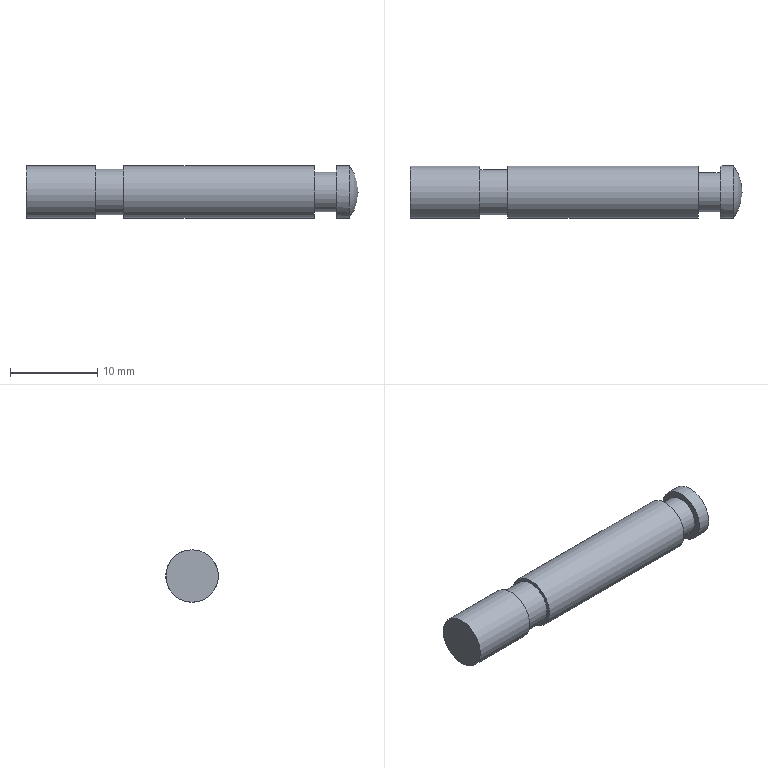Component | NX | SUPPORT_STUD | 1 solid | 11 faces | box 38 x 6 x 6 mm | volume 1007 mm3 | cylinder 5 | plane 5 | sphere 1 | commonest cylinder face diameters 6 x3 4.5 x1 5.188 x1
STEP:
#1=CARTESIAN_POINT('',(0.,0.,0.));
#2=DIRECTION('',(0.,0.,1.));
#3=DIRECTION('',(1.,0.,0.));
#4=AXIS2_PLACEMENT_3D('',#1,#2,#3);
#5=CARTESIAN_POINT('',(-18.8,-52.,-54.));
#6=VERTEX_POINT('',#5);
#7=CARTESIAN_POINT('',(-18.8,-52.,-57.));
#8=DIRECTION('',(1.,0.,-0.));
#9=DIRECTION('',(0.,0.,1.));
#10=AXIS2_PLACEMENT_3D('',#7,#8,#9);
#11=CIRCLE('',#10,3.);
#12=CARTESIAN_POINT('',(-30.,-52.,-57.));
#13=DIRECTION('',(1.,0.,0.));
#14=DIRECTION('',(0.,0.,1.));
#15=AXIS2_PLACEMENT_3D('',#12,#13,#14);
#16=CYLINDRICAL_SURFACE('',#15,3.);
#17=CARTESIAN_POINT('',(0.,11.2));
#18=DIRECTION('',(1.,0.));
#19=VECTOR('',#18,1.);
#20=LINE('',#17,#19);
#21=(GEOMETRIC_REPRESENTATION_CONTEXT(2)PARAMETRIC_REPRESENTATION_CONTEXT()REPRESENTATION_CONTEXT('',''));
#22=DEFINITIONAL_REPRESENTATION('',(#20),#21);
#23=PCURVE('',#16,#22);
#24=CARTESIAN_POINT('',(-18.8,-52.,-57.));
#25=DIRECTION('',(1.,0.,-0.));
#26=DIRECTION('',(0.,-1.,0.));
#27=AXIS2_PLACEMENT_3D('',#24,#25,#26);
#28=PLANE('',#27);
#29=CARTESIAN_POINT('',(0.,0.));
#30=DIRECTION('',(0.,-1.));
#31=AXIS2_PLACEMENT_2D('',#29,#30);
#32=CIRCLE('',#31,3.);
#33=(GEOMETRIC_REPRESENTATION_CONTEXT(2)PARAMETRIC_REPRESENTATION_CONTEXT()REPRESENTATION_CONTEXT('',''));
#34=DEFINITIONAL_REPRESENTATION('',(#32),#33);
#35=PCURVE('',#28,#34);
#36=SURFACE_CURVE('',#11,(#23,#35),.PCURVE_S1.);
#37=EDGE_CURVE('',#6,#6,#36,.T.);
#38=ORIENTED_EDGE('',*,*,#37,.T.);
#39=CARTESIAN_POINT('',(3.,-52.,-54.));
#40=VERTEX_POINT('',#39);
#41=CARTESIAN_POINT('',(-18.8,-52.,-54.));
#42=CARTESIAN_POINT('',(3.,-52.,-54.));
#43=B_SPLINE_CURVE_WITH_KNOTS('',1,(#41,#42),.UNSPECIFIED.,.F.,.F.,(2,2),(11.2,33.),.PIECEWISE_BEZIER_KNOTS.);
#44=CARTESIAN_POINT('',(6.283,0.));
#45=DIRECTION('',(0.,1.));
#46=VECTOR('',#45,1.);
#47=LINE('',#44,#46);
#48=(GEOMETRIC_REPRESENTATION_CONTEXT(2)PARAMETRIC_REPRESENTATION_CONTEXT()REPRESENTATION_CONTEXT('',''));
#49=DEFINITIONAL_REPRESENTATION('',(#47),#48);
#50=PCURVE('',#16,#49);
#51=CARTESIAN_POINT('',(0.,0.));
#52=DIRECTION('',(0.,1.));
#53=VECTOR('',#52,1.);
#54=LINE('',#51,#53);
#55=(GEOMETRIC_REPRESENTATION_CONTEXT(2)PARAMETRIC_REPRESENTATION_CONTEXT()REPRESENTATION_CONTEXT('',''));
#56=DEFINITIONAL_REPRESENTATION('',(#54),#55);
#57=PCURVE('',#16,#56);
#58=SEAM_CURVE('',#43,(#50,#57),.PCURVE_S1.);
#59=EDGE_CURVE('',#6,#40,#58,.T.);
#60=ORIENTED_EDGE('',*,*,#59,.T.);
#61=CARTESIAN_POINT('',(3.,-52.,-57.));
#62=DIRECTION('',(1.,0.,0.));
#63=DIRECTION('',(0.,0.,1.));
#64=AXIS2_PLACEMENT_3D('',#61,#62,#63);
#65=CIRCLE('',#64,3.);
#66=CARTESIAN_POINT('',(0.,33.));
#67=DIRECTION('',(1.,0.));
#68=VECTOR('',#67,1.);
#69=LINE('',#66,#68);
#70=(GEOMETRIC_REPRESENTATION_CONTEXT(2)PARAMETRIC_REPRESENTATION_CONTEXT()REPRESENTATION_CONTEXT('',''));
#71=DEFINITIONAL_REPRESENTATION('',(#69),#70);
#72=PCURVE('',#16,#71);
#73=CARTESIAN_POINT('',(3.,-52.,-57.));
#74=DIRECTION('',(1.,0.,0.));
#75=DIRECTION('',(0.,0.,1.));
#76=AXIS2_PLACEMENT_3D('',#73,#74,#75);
#77=PLANE('',#76);
#78=CARTESIAN_POINT('',(0.,0.));
#79=DIRECTION('',(1.,0.));
#80=AXIS2_PLACEMENT_2D('',#78,#79);
#81=CIRCLE('',#80,3.);
#82=(GEOMETRIC_REPRESENTATION_CONTEXT(2)PARAMETRIC_REPRESENTATION_CONTEXT()REPRESENTATION_CONTEXT('',''));
#83=DEFINITIONAL_REPRESENTATION('',(#81),#82);
#84=PCURVE('',#77,#83);
#85=SURFACE_CURVE('',#65,(#72,#84),.PCURVE_S1.);
#86=EDGE_CURVE('',#40,#40,#85,.T.);
#87=ORIENTED_EDGE('',*,*,#86,.F.);
#88=ORIENTED_EDGE('',*,*,#59,.F.);
#89=EDGE_LOOP('',(#38,#60,#87,#88));
#90=FACE_BOUND('',#89,.T.);
#91=ADVANCED_FACE('',(#90),#16,.T.);
#92=CARTESIAN_POINT('',(3.,-52.,-54.75));
#93=VERTEX_POINT('',#92);
#94=CARTESIAN_POINT('',(3.,-52.,-57.));
#95=DIRECTION('',(-1.,0.,0.));
#96=DIRECTION('',(0.,0.,1.));
#97=AXIS2_PLACEMENT_3D('',#94,#95,#96);
#98=CIRCLE('',#97,2.25);
#99=CARTESIAN_POINT('',(2.25,0.));
#100=CARTESIAN_POINT('',(2.25,-3.897));
#101=CARTESIAN_POINT('',(-1.125,-1.949));
#102=CARTESIAN_POINT('',(-4.5,-0.));
#103=CARTESIAN_POINT('',(-1.125,1.949));
#104=CARTESIAN_POINT('',(2.25,3.897));
#105=CARTESIAN_POINT('',(2.25,0.));
#106=(BOUNDED_CURVE()B_SPLINE_CURVE(2,(#99,#100,#101,#102,#103,#104,#105),.UNSPECIFIED.,.T.,.F.)B_SPLINE_CURVE_WITH_KNOTS((1,2,2,2,2,1),(-2.094,0.,2.094,4.189,6.283,8.378),.UNSPECIFIED.)CURVE()GEOMETRIC_REPRESENTATION_ITEM()RATIONAL_B_SPLINE_CURVE((1.,0.5,1.,0.5,1.,0.5,1.))REPRESENTATION_ITEM(''));
#107=(GEOMETRIC_REPRESENTATION_CONTEXT(2)PARAMETRIC_REPRESENTATION_CONTEXT()REPRESENTATION_CONTEXT('',''));
#108=DEFINITIONAL_REPRESENTATION('',(#106),#107);
#109=PCURVE('',#77,#108);
#110=CARTESIAN_POINT('',(-3.75,-52.,-57.));
#111=DIRECTION('',(1.,0.,0.));
#112=DIRECTION('',(0.,0.,1.));
#113=AXIS2_PLACEMENT_3D('',#110,#111,#112);
#114=CYLINDRICAL_SURFACE('',#113,2.25);
#115=CARTESIAN_POINT('',(6.283,6.75));
#116=DIRECTION('',(-1.,0.));
#117=VECTOR('',#116,1.);
#118=LINE('',#115,#117);
#119=(GEOMETRIC_REPRESENTATION_CONTEXT(2)PARAMETRIC_REPRESENTATION_CONTEXT()REPRESENTATION_CONTEXT('',''));
#120=DEFINITIONAL_REPRESENTATION('',(#118),#119);
#121=PCURVE('',#114,#120);
#122=SURFACE_CURVE('',#98,(#109,#121),.PCURVE_S1.);
#123=EDGE_CURVE('',#93,#93,#122,.T.);
#124=ORIENTED_EDGE('',*,*,#123,.T.);
#125=EDGE_LOOP('',(#124));
#126=FACE_BOUND('',#125,.T.);
#127=ORIENTED_EDGE('',*,*,#86,.T.);
#128=EDGE_LOOP('',(#127));
#129=FACE_BOUND('',#128,.T.);
#130=ADVANCED_FACE('',(#126,#129),#77,.T.);
#131=CARTESIAN_POINT('',(5.5,-52.,-54.75));
#132=VERTEX_POINT('',#131);
#133=CARTESIAN_POINT('',(5.5,-52.,-57.));
#134=DIRECTION('',(-1.,0.,0.));
#135=DIRECTION('',(0.,0.,1.));
#136=AXIS2_PLACEMENT_3D('',#133,#134,#135);
#137=CIRCLE('',#136,2.25);
#138=CARTESIAN_POINT('',(5.5,-52.,-57.));
#139=DIRECTION('',(1.,0.,0.));
#140=DIRECTION('',(0.,0.,1.));
#141=AXIS2_PLACEMENT_3D('',#138,#139,#140);
#142=PLANE('',#141);
#143=CARTESIAN_POINT('',(2.25,0.));
#144=CARTESIAN_POINT('',(2.25,-3.897));
#145=CARTESIAN_POINT('',(-1.125,-1.949));
#146=CARTESIAN_POINT('',(-4.5,-0.));
#147=CARTESIAN_POINT('',(-1.125,1.949));
#148=CARTESIAN_POINT('',(2.25,3.897));
#149=CARTESIAN_POINT('',(2.25,0.));
#150=(BOUNDED_CURVE()B_SPLINE_CURVE(2,(#143,#144,#145,#146,#147,#148,#149),.UNSPECIFIED.,.T.,.F.)B_SPLINE_CURVE_WITH_KNOTS((1,2,2,2,2,1),(-2.094,0.,2.094,4.189,6.283,8.378),.UNSPECIFIED.)CURVE()GEOMETRIC_REPRESENTATION_ITEM()RATIONAL_B_SPLINE_CURVE((1.,0.5,1.,0.5,1.,0.5,1.))REPRESENTATION_ITEM(''));
#151=(GEOMETRIC_REPRESENTATION_CONTEXT(2)PARAMETRIC_REPRESENTATION_CONTEXT()REPRESENTATION_CONTEXT('',''));
#152=DEFINITIONAL_REPRESENTATION('',(#150),#151);
#153=PCURVE('',#142,#152);
#154=CARTESIAN_POINT('',(6.283,9.25));
#155=DIRECTION('',(-1.,0.));
#156=VECTOR('',#155,1.);
#157=LINE('',#154,#156);
#158=(GEOMETRIC_REPRESENTATION_CONTEXT(2)PARAMETRIC_REPRESENTATION_CONTEXT()REPRESENTATION_CONTEXT('',''));
#159=DEFINITIONAL_REPRESENTATION('',(#157),#158);
#160=PCURVE('',#114,#159);
#161=SURFACE_CURVE('',#137,(#153,#160),.PCURVE_S1.);
#162=EDGE_CURVE('',#132,#132,#161,.T.);
#163=ORIENTED_EDGE('',*,*,#162,.F.);
#164=EDGE_LOOP('',(#163));
#165=FACE_BOUND('',#164,.T.);
#166=CARTESIAN_POINT('',(5.5,-52.,-54.));
#167=VERTEX_POINT('',#166);
#168=CARTESIAN_POINT('',(5.5,-52.,-57.));
#169=DIRECTION('',(1.,0.,0.));
#170=DIRECTION('',(0.,0.,1.));
#171=AXIS2_PLACEMENT_3D('',#168,#169,#170);
#172=CIRCLE('',#171,3.);
#173=CARTESIAN_POINT('',(0.,0.));
#174=DIRECTION('',(1.,0.));
#175=AXIS2_PLACEMENT_2D('',#173,#174);
#176=CIRCLE('',#175,3.);
#177=(GEOMETRIC_REPRESENTATION_CONTEXT(2)PARAMETRIC_REPRESENTATION_CONTEXT()REPRESENTATION_CONTEXT('',''));
#178=DEFINITIONAL_REPRESENTATION('',(#176),#177);
#179=PCURVE('',#142,#178);
#180=CARTESIAN_POINT('',(-30.,-52.,-57.));
#181=DIRECTION('',(1.,0.,0.));
#182=DIRECTION('',(0.,0.,1.));
#183=AXIS2_PLACEMENT_3D('',#180,#181,#182);
#184=CYLINDRICAL_SURFACE('',#183,3.);
#185=CARTESIAN_POINT('',(0.,35.5));
#186=DIRECTION('',(1.,0.));
#187=VECTOR('',#186,1.);
#188=LINE('',#185,#187);
#189=(GEOMETRIC_REPRESENTATION_CONTEXT(2)PARAMETRIC_REPRESENTATION_CONTEXT()REPRESENTATION_CONTEXT('',''));
#190=DEFINITIONAL_REPRESENTATION('',(#188),#189);
#191=PCURVE('',#184,#190);
#192=SURFACE_CURVE('',#172,(#179,#191),.PCURVE_S1.);
#193=EDGE_CURVE('',#167,#167,#192,.T.);
#194=ORIENTED_EDGE('',*,*,#193,.F.);
#195=EDGE_LOOP('',(#194));
#196=FACE_BOUND('',#195,.T.);
#197=ADVANCED_FACE('',(#165,#196),#142,.F.);
#198=ORIENTED_EDGE('',*,*,#162,.T.);
#199=CARTESIAN_POINT('',(3.,-52.,-54.75));
#200=CARTESIAN_POINT('',(5.5,-52.,-54.75));
#201=B_SPLINE_CURVE_WITH_KNOTS('',1,(#199,#200),.UNSPECIFIED.,.F.,.F.,(2,2),(6.75,9.25),.PIECEWISE_BEZIER_KNOTS.);
#202=CARTESIAN_POINT('',(0.,0.));
#203=DIRECTION('',(0.,1.));
#204=VECTOR('',#203,1.);
#205=LINE('',#202,#204);
#206=(GEOMETRIC_REPRESENTATION_CONTEXT(2)PARAMETRIC_REPRESENTATION_CONTEXT()REPRESENTATION_CONTEXT('',''));
#207=DEFINITIONAL_REPRESENTATION('',(#205),#206);
#208=PCURVE('',#114,#207);
#209=CARTESIAN_POINT('',(6.283,0.));
#210=DIRECTION('',(0.,1.));
#211=VECTOR('',#210,1.);
#212=LINE('',#209,#211);
#213=(GEOMETRIC_REPRESENTATION_CONTEXT(2)PARAMETRIC_REPRESENTATION_CONTEXT()REPRESENTATION_CONTEXT('',''));
#214=DEFINITIONAL_REPRESENTATION('',(#212),#213);
#215=PCURVE('',#114,#214);
#216=SEAM_CURVE('',#201,(#208,#215),.PCURVE_S1.);
#217=EDGE_CURVE('',#93,#132,#216,.T.);
#218=ORIENTED_EDGE('',*,*,#217,.F.);
#219=ORIENTED_EDGE('',*,*,#123,.F.);
#220=ORIENTED_EDGE('',*,*,#217,.T.);
#221=EDGE_LOOP('',(#198,#218,#219,#220));
#222=FACE_BOUND('',#221,.T.);
#223=ADVANCED_FACE('',(#222),#114,.T.);
#224=CARTESIAN_POINT('',(7.,-52.,-54.));
#225=VERTEX_POINT('',#224);
#226=CARTESIAN_POINT('',(7.,-49.,-57.));
#227=VERTEX_POINT('',#226);
#228=CARTESIAN_POINT('',(7.,-52.,-57.));
#229=DIRECTION('',(1.,0.,0.));
#230=DIRECTION('',(0.,0.,1.));
#231=AXIS2_PLACEMENT_3D('',#228,#229,#230);
#232=CIRCLE('',#231,3.);
#233=CARTESIAN_POINT('',(3.,-52.,-57.));
#234=DIRECTION('',(1.,0.,0.));
#235=DIRECTION('',(0.,1.,0.));
#236=AXIS2_PLACEMENT_3D('',#233,#234,#235);
#237=SPHERICAL_SURFACE('',#236,5.);
#238=CARTESIAN_POINT('',(1.571,0.9273));
#239=CARTESIAN_POINT('',(1.666,0.9273));
#240=CARTESIAN_POINT('',(1.856,0.9273));
#241=CARTESIAN_POINT('',(2.142,0.9273));
#242=CARTESIAN_POINT('',(2.428,0.9273));
#243=CARTESIAN_POINT('',(2.713,0.9273));
#244=CARTESIAN_POINT('',(2.999,0.9273));
#245=CARTESIAN_POINT('',(3.284,0.9273));
#246=CARTESIAN_POINT('',(3.57,0.9273));
#247=CARTESIAN_POINT('',(3.856,0.9273));
#248=CARTESIAN_POINT('',(4.141,0.9273));
#249=CARTESIAN_POINT('',(4.427,0.9273));
#250=CARTESIAN_POINT('',(4.712,0.9273));
#251=CARTESIAN_POINT('',(4.998,0.9273));
#252=CARTESIAN_POINT('',(5.284,0.9273));
#253=CARTESIAN_POINT('',(5.569,0.9273));
#254=CARTESIAN_POINT('',(5.855,0.9273));
#255=CARTESIAN_POINT('',(6.14,0.9273));
#256=CARTESIAN_POINT('',(6.426,0.9273));
#257=CARTESIAN_POINT('',(6.712,0.9273));
#258=CARTESIAN_POINT('',(6.997,0.9273));
#259=CARTESIAN_POINT('',(7.283,0.9273));
#260=CARTESIAN_POINT('',(7.568,0.9273));
#261=CARTESIAN_POINT('',(7.759,0.9273));
#262=CARTESIAN_POINT('',(7.854,0.9273));
#263=B_SPLINE_CURVE_WITH_KNOTS('',3,(#238,#239,#240,#241,#242,#243,#244,#245,#246,#247,#248,#249,#250,#251,#252,#253,#254,#255,#256,#257,#258,#259,#260,#261,#262),.UNSPECIFIED.,.F.,.F.,(4,1,1,1,1,1,1,1,1,1,1,1,1,1,1,1,1,1,1,1,1,1,4),(0.,0.2856,0.5712,0.8568,1.142,1.428,1.714,1.999,2.285,2.57,2.856,3.142,3.427,3.713,3.998,4.284,4.57,4.855,5.141,5.426,5.712,5.998,6.283),.QUASI_UNIFORM_KNOTS.);
#264=(GEOMETRIC_REPRESENTATION_CONTEXT(2)PARAMETRIC_REPRESENTATION_CONTEXT()REPRESENTATION_CONTEXT('',''));
#265=DEFINITIONAL_REPRESENTATION('',(#263),#264);
#266=PCURVE('',#237,#265);
#267=CARTESIAN_POINT('',(0.,37.));
#268=DIRECTION('',(1.,0.));
#269=VECTOR('',#268,1.);
#270=LINE('',#267,#269);
#271=(GEOMETRIC_REPRESENTATION_CONTEXT(2)PARAMETRIC_REPRESENTATION_CONTEXT()REPRESENTATION_CONTEXT('',''));
#272=DEFINITIONAL_REPRESENTATION('',(#270),#271);
#273=PCURVE('',#184,#272);
#274=SURFACE_CURVE('',#232,(#266,#273),.PCURVE_S1.);
#275=EDGE_CURVE('',#225,#227,#274,.T.);
#276=ORIENTED_EDGE('',*,*,#275,.T.);
#277=CARTESIAN_POINT('',(8.,-52.,-57.));
#278=VERTEX_POINT('',#277);
#279=CARTESIAN_POINT('',(7.,-49.,-57.));
#280=CARTESIAN_POINT('',(7.386,-49.515,-57.));
#281=CARTESIAN_POINT('',(7.689,-50.092,-57.));
#282=CARTESIAN_POINT('',(7.896,-50.713,-57.));
#283=CARTESIAN_POINT('',(8.,-51.356,-57.));
#284=CARTESIAN_POINT('',(8.,-52.,-57.));
#285=B_SPLINE_CURVE_WITH_KNOTS('',5,(#279,#280,#281,#282,#283,#284),.UNSPECIFIED.,.F.,.F.,(6,6),(0.9273,1.571),.PIECEWISE_BEZIER_KNOTS.);
#286=CARTESIAN_POINT('',(6.283,0.));
#287=DIRECTION('',(0.,1.));
#288=VECTOR('',#287,1.);
#289=LINE('',#286,#288);
#290=(GEOMETRIC_REPRESENTATION_CONTEXT(2)PARAMETRIC_REPRESENTATION_CONTEXT()REPRESENTATION_CONTEXT('',''));
#291=DEFINITIONAL_REPRESENTATION('',(#289),#290);
#292=PCURVE('',#237,#291);
#293=CARTESIAN_POINT('',(0.,0.));
#294=DIRECTION('',(0.,1.));
#295=VECTOR('',#294,1.);
#296=LINE('',#293,#295);
#297=(GEOMETRIC_REPRESENTATION_CONTEXT(2)PARAMETRIC_REPRESENTATION_CONTEXT()REPRESENTATION_CONTEXT('',''));
#298=DEFINITIONAL_REPRESENTATION('',(#296),#297);
#299=PCURVE('',#237,#298);
#300=SEAM_CURVE('',#285,(#292,#299),.PCURVE_S1.);
#301=EDGE_CURVE('',#227,#278,#300,.T.);
#302=ORIENTED_EDGE('',*,*,#301,.T.);
#303=ORIENTED_EDGE('',*,*,#301,.F.);
#304=CARTESIAN_POINT('',(7.,-52.,-57.));
#305=DIRECTION('',(1.,0.,0.));
#306=DIRECTION('',(0.,0.,1.));
#307=AXIS2_PLACEMENT_3D('',#304,#305,#306);
#308=CIRCLE('',#307,3.);
#309=CARTESIAN_POINT('',(-4.712,0.9273));
#310=CARTESIAN_POINT('',(-4.617,0.9273));
#311=CARTESIAN_POINT('',(-4.427,0.9273));
#312=CARTESIAN_POINT('',(-4.141,0.9273));
#313=CARTESIAN_POINT('',(-3.856,0.9273));
#314=CARTESIAN_POINT('',(-3.57,0.9273));
#315=CARTESIAN_POINT('',(-3.284,0.9273));
#316=CARTESIAN_POINT('',(-2.999,0.9273));
#317=CARTESIAN_POINT('',(-2.713,0.9273));
#318=CARTESIAN_POINT('',(-2.428,0.9273));
#319=CARTESIAN_POINT('',(-2.142,0.9273));
#320=CARTESIAN_POINT('',(-1.856,0.9273));
#321=CARTESIAN_POINT('',(-1.571,0.9273));
#322=CARTESIAN_POINT('',(-1.285,0.9273));
#323=CARTESIAN_POINT('',(-0.9996,0.9273));
#324=CARTESIAN_POINT('',(-0.714,0.9273));
#325=CARTESIAN_POINT('',(-0.4284,0.9273));
#326=CARTESIAN_POINT('',(-0.1428,0.9273));
#327=CARTESIAN_POINT('',(0.1428,0.9273));
#328=CARTESIAN_POINT('',(0.4284,0.9273));
#329=CARTESIAN_POINT('',(0.714,0.9273));
#330=CARTESIAN_POINT('',(0.9996,0.9273));
#331=CARTESIAN_POINT('',(1.285,0.9273));
#332=CARTESIAN_POINT('',(1.476,0.9273));
#333=CARTESIAN_POINT('',(1.571,0.9273));
#334=B_SPLINE_CURVE_WITH_KNOTS('',3,(#309,#310,#311,#312,#313,#314,#315,#316,#317,#318,#319,#320,#321,#322,#323,#324,#325,#326,#327,#328,#329,#330,#331,#332,#333),.UNSPECIFIED.,.F.,.F.,(4,1,1,1,1,1,1,1,1,1,1,1,1,1,1,1,1,1,1,1,1,1,4),(0.,0.2856,0.5712,0.8568,1.142,1.428,1.714,1.999,2.285,2.57,2.856,3.142,3.427,3.713,3.998,4.284,4.57,4.855,5.141,5.426,5.712,5.998,6.283),.QUASI_UNIFORM_KNOTS.);
#335=(GEOMETRIC_REPRESENTATION_CONTEXT(2)PARAMETRIC_REPRESENTATION_CONTEXT()REPRESENTATION_CONTEXT('',''));
#336=DEFINITIONAL_REPRESENTATION('',(#334),#335);
#337=PCURVE('',#237,#336);
#338=CARTESIAN_POINT('',(0.,37.));
#339=DIRECTION('',(1.,0.));
#340=VECTOR('',#339,1.);
#341=LINE('',#338,#340);
#342=(GEOMETRIC_REPRESENTATION_CONTEXT(2)PARAMETRIC_REPRESENTATION_CONTEXT()REPRESENTATION_CONTEXT('',''));
#343=DEFINITIONAL_REPRESENTATION('',(#341),#342);
#344=PCURVE('',#184,#343);
#345=SURFACE_CURVE('',#308,(#337,#344),.PCURVE_S1.);
#346=EDGE_CURVE('',#227,#225,#345,.T.);
#347=ORIENTED_EDGE('',*,*,#346,.T.);
#348=EDGE_LOOP('',(#276,#302,#303,#347));
#349=FACE_BOUND('',#348,.T.);
#350=ADVANCED_FACE('',(#349),#237,.T.);
#351=ORIENTED_EDGE('',*,*,#193,.T.);
#352=CARTESIAN_POINT('',(5.5,-52.,-54.));
#353=CARTESIAN_POINT('',(7.,-52.,-54.));
#354=B_SPLINE_CURVE_WITH_KNOTS('',1,(#352,#353),.UNSPECIFIED.,.F.,.F.,(2,2),(35.5,37.),.PIECEWISE_BEZIER_KNOTS.);
#355=CARTESIAN_POINT('',(6.283,0.));
#356=DIRECTION('',(0.,1.));
#357=VECTOR('',#356,1.);
#358=LINE('',#355,#357);
#359=(GEOMETRIC_REPRESENTATION_CONTEXT(2)PARAMETRIC_REPRESENTATION_CONTEXT()REPRESENTATION_CONTEXT('',''));
#360=DEFINITIONAL_REPRESENTATION('',(#358),#359);
#361=PCURVE('',#184,#360);
#362=CARTESIAN_POINT('',(0.,0.));
#363=DIRECTION('',(0.,1.));
#364=VECTOR('',#363,1.);
#365=LINE('',#362,#364);
#366=(GEOMETRIC_REPRESENTATION_CONTEXT(2)PARAMETRIC_REPRESENTATION_CONTEXT()REPRESENTATION_CONTEXT('',''));
#367=DEFINITIONAL_REPRESENTATION('',(#365),#366);
#368=PCURVE('',#184,#367);
#369=SEAM_CURVE('',#354,(#361,#368),.PCURVE_S1.);
#370=EDGE_CURVE('',#167,#225,#369,.T.);
#371=ORIENTED_EDGE('',*,*,#370,.T.);
#372=ORIENTED_EDGE('',*,*,#346,.F.);
#373=ORIENTED_EDGE('',*,*,#275,.F.);
#374=ORIENTED_EDGE('',*,*,#370,.F.);
#375=EDGE_LOOP('',(#351,#371,#372,#373,#374));
#376=FACE_BOUND('',#375,.T.);
#377=ADVANCED_FACE('',(#376),#184,.T.);
#378=CARTESIAN_POINT('',(-18.8,-52.,-54.406));
#379=VERTEX_POINT('',#378);
#380=CARTESIAN_POINT('',(-18.8,-52.,-57.));
#381=DIRECTION('',(1.,0.,-0.));
#382=DIRECTION('',(0.,0.,1.));
#383=AXIS2_PLACEMENT_3D('',#380,#381,#382);
#384=CIRCLE('',#383,2.594);
#385=CARTESIAN_POINT('',(0.,0.));
#386=DIRECTION('',(0.,-1.));
#387=AXIS2_PLACEMENT_2D('',#385,#386);
#388=CIRCLE('',#387,2.594);
#389=(GEOMETRIC_REPRESENTATION_CONTEXT(2)PARAMETRIC_REPRESENTATION_CONTEXT()REPRESENTATION_CONTEXT('',''));
#390=DEFINITIONAL_REPRESENTATION('',(#388),#389);
#391=PCURVE('',#28,#390);
#392=CARTESIAN_POINT('',(-22.,-52.,-57.));
#393=DIRECTION('',(1.,0.,0.));
#394=DIRECTION('',(0.,0.,1.));
#395=AXIS2_PLACEMENT_3D('',#392,#393,#394);
#396=CYLINDRICAL_SURFACE('',#395,2.594);
#397=CARTESIAN_POINT('',(0.,3.2));
#398=DIRECTION('',(1.,0.));
#399=VECTOR('',#398,1.);
#400=LINE('',#397,#399);
#401=(GEOMETRIC_REPRESENTATION_CONTEXT(2)PARAMETRIC_REPRESENTATION_CONTEXT()REPRESENTATION_CONTEXT('',''));
#402=DEFINITIONAL_REPRESENTATION('',(#400),#401);
#403=PCURVE('',#396,#402);
#404=SURFACE_CURVE('',#384,(#391,#403),.PCURVE_S1.);
#405=EDGE_CURVE('',#379,#379,#404,.T.);
#406=ORIENTED_EDGE('',*,*,#405,.T.);
#407=EDGE_LOOP('',(#406));
#408=FACE_BOUND('',#407,.T.);
#409=ORIENTED_EDGE('',*,*,#37,.F.);
#410=EDGE_LOOP('',(#409));
#411=FACE_BOUND('',#410,.T.);
#412=ADVANCED_FACE('',(#408,#411),#28,.F.);
#413=CARTESIAN_POINT('',(-22.,-52.,-54.406));
#414=VERTEX_POINT('',#413);
#415=CARTESIAN_POINT('',(-22.,-52.,-57.));
#416=DIRECTION('',(1.,0.,0.));
#417=DIRECTION('',(0.,0.,1.));
#418=AXIS2_PLACEMENT_3D('',#415,#416,#417);
#419=CIRCLE('',#418,2.594);
#420=CARTESIAN_POINT('',(-22.,-52.,-57.));
#421=DIRECTION('',(1.,0.,0.));
#422=DIRECTION('',(0.,-1.,0.));
#423=AXIS2_PLACEMENT_3D('',#420,#421,#422);
#424=PLANE('',#423);
#425=CARTESIAN_POINT('',(0.,0.));
#426=DIRECTION('',(0.,-1.));
#427=AXIS2_PLACEMENT_2D('',#425,#426);
#428=CIRCLE('',#427,2.594);
#429=(GEOMETRIC_REPRESENTATION_CONTEXT(2)PARAMETRIC_REPRESENTATION_CONTEXT()REPRESENTATION_CONTEXT('',''));
#430=DEFINITIONAL_REPRESENTATION('',(#428),#429);
#431=PCURVE('',#424,#430);
#432=CARTESIAN_POINT('',(0.,0.));
#433=DIRECTION('',(1.,0.));
#434=VECTOR('',#433,1.);
#435=LINE('',#432,#434);
#436=(GEOMETRIC_REPRESENTATION_CONTEXT(2)PARAMETRIC_REPRESENTATION_CONTEXT()REPRESENTATION_CONTEXT('',''));
#437=DEFINITIONAL_REPRESENTATION('',(#435),#436);
#438=PCURVE('',#396,#437);
#439=SURFACE_CURVE('',#419,(#431,#438),.PCURVE_S1.);
#440=EDGE_CURVE('',#414,#414,#439,.T.);
#441=ORIENTED_EDGE('',*,*,#440,.F.);
#442=EDGE_LOOP('',(#441));
#443=FACE_BOUND('',#442,.T.);
#444=CARTESIAN_POINT('',(-22.,-52.,-54.));
#445=VERTEX_POINT('',#444);
#446=CARTESIAN_POINT('',(-22.,-52.,-57.));
#447=DIRECTION('',(1.,0.,0.));
#448=DIRECTION('',(0.,0.,1.));
#449=AXIS2_PLACEMENT_3D('',#446,#447,#448);
#450=CIRCLE('',#449,3.);
#451=CARTESIAN_POINT('',(0.,0.));
#452=DIRECTION('',(0.,-1.));
#453=AXIS2_PLACEMENT_2D('',#451,#452);
#454=CIRCLE('',#453,3.);
#455=(GEOMETRIC_REPRESENTATION_CONTEXT(2)PARAMETRIC_REPRESENTATION_CONTEXT()REPRESENTATION_CONTEXT('',''));
#456=DEFINITIONAL_REPRESENTATION('',(#454),#455);
#457=PCURVE('',#424,#456);
#458=CARTESIAN_POINT('',(-30.,-52.,-57.));
#459=DIRECTION('',(1.,0.,0.));
#460=DIRECTION('',(0.,0.,1.));
#461=AXIS2_PLACEMENT_3D('',#458,#459,#460);
#462=CYLINDRICAL_SURFACE('',#461,3.);
#463=CARTESIAN_POINT('',(0.,8.));
#464=DIRECTION('',(1.,0.));
#465=VECTOR('',#464,1.);
#466=LINE('',#463,#465);
#467=(GEOMETRIC_REPRESENTATION_CONTEXT(2)PARAMETRIC_REPRESENTATION_CONTEXT()REPRESENTATION_CONTEXT('',''));
#468=DEFINITIONAL_REPRESENTATION('',(#466),#467);
#469=PCURVE('',#462,#468);
#470=SURFACE_CURVE('',#450,(#457,#469),.PCURVE_S1.);
#471=EDGE_CURVE('',#445,#445,#470,.T.);
#472=ORIENTED_EDGE('',*,*,#471,.T.);
#473=EDGE_LOOP('',(#472));
#474=FACE_BOUND('',#473,.T.);
#475=ADVANCED_FACE('',(#443,#474),#424,.T.);
#476=ORIENTED_EDGE('',*,*,#440,.T.);
#477=CARTESIAN_POINT('',(-22.,-52.,-54.406));
#478=CARTESIAN_POINT('',(-18.8,-52.,-54.406));
#479=B_SPLINE_CURVE_WITH_KNOTS('',1,(#477,#478),.UNSPECIFIED.,.F.,.F.,(2,2),(0.,3.2),.PIECEWISE_BEZIER_KNOTS.);
#480=CARTESIAN_POINT('',(6.283,0.));
#481=DIRECTION('',(0.,1.));
#482=VECTOR('',#481,1.);
#483=LINE('',#480,#482);
#484=(GEOMETRIC_REPRESENTATION_CONTEXT(2)PARAMETRIC_REPRESENTATION_CONTEXT()REPRESENTATION_CONTEXT('',''));
#485=DEFINITIONAL_REPRESENTATION('',(#483),#484);
#486=PCURVE('',#396,#485);
#487=CARTESIAN_POINT('',(0.,0.));
#488=DIRECTION('',(0.,1.));
#489=VECTOR('',#488,1.);
#490=LINE('',#487,#489);
#491=(GEOMETRIC_REPRESENTATION_CONTEXT(2)PARAMETRIC_REPRESENTATION_CONTEXT()REPRESENTATION_CONTEXT('',''));
#492=DEFINITIONAL_REPRESENTATION('',(#490),#491);
#493=PCURVE('',#396,#492);
#494=SEAM_CURVE('',#479,(#486,#493),.PCURVE_S1.);
#495=EDGE_CURVE('',#414,#379,#494,.T.);
#496=ORIENTED_EDGE('',*,*,#495,.T.);
#497=ORIENTED_EDGE('',*,*,#405,.F.);
#498=ORIENTED_EDGE('',*,*,#495,.F.);
#499=EDGE_LOOP('',(#476,#496,#497,#498));
#500=FACE_BOUND('',#499,.T.);
#501=ADVANCED_FACE('',(#500),#396,.T.);
#502=CARTESIAN_POINT('',(-30.,-52.,-54.));
#503=VERTEX_POINT('',#502);
#504=CARTESIAN_POINT('',(-30.,-52.,-57.));
#505=DIRECTION('',(1.,0.,0.));
#506=DIRECTION('',(0.,0.,1.));
#507=AXIS2_PLACEMENT_3D('',#504,#505,#506);
#508=CIRCLE('',#507,3.);
#509=CARTESIAN_POINT('',(-30.,-52.,-57.));
#510=DIRECTION('',(1.,0.,0.));
#511=DIRECTION('',(0.,0.,1.));
#512=AXIS2_PLACEMENT_3D('',#509,#510,#511);
#513=PLANE('',#512);
#514=CARTESIAN_POINT('',(0.,0.));
#515=DIRECTION('',(1.,0.));
#516=AXIS2_PLACEMENT_2D('',#514,#515);
#517=CIRCLE('',#516,3.);
#518=(GEOMETRIC_REPRESENTATION_CONTEXT(2)PARAMETRIC_REPRESENTATION_CONTEXT()REPRESENTATION_CONTEXT('',''));
#519=DEFINITIONAL_REPRESENTATION('',(#517),#518);
#520=PCURVE('',#513,#519);
#521=CARTESIAN_POINT('',(0.,0.));
#522=DIRECTION('',(1.,0.));
#523=VECTOR('',#522,1.);
#524=LINE('',#521,#523);
#525=(GEOMETRIC_REPRESENTATION_CONTEXT(2)PARAMETRIC_REPRESENTATION_CONTEXT()REPRESENTATION_CONTEXT('',''));
#526=DEFINITIONAL_REPRESENTATION('',(#524),#525);
#527=PCURVE('',#462,#526);
#528=SURFACE_CURVE('',#508,(#520,#527),.PCURVE_S1.);
#529=EDGE_CURVE('',#503,#503,#528,.T.);
#530=ORIENTED_EDGE('',*,*,#529,.F.);
#531=EDGE_LOOP('',(#530));
#532=FACE_BOUND('',#531,.T.);
#533=ADVANCED_FACE('',(#532),#513,.F.);
#534=ORIENTED_EDGE('',*,*,#529,.T.);
#535=CARTESIAN_POINT('',(-30.,-52.,-54.));
#536=CARTESIAN_POINT('',(-22.,-52.,-54.));
#537=B_SPLINE_CURVE_WITH_KNOTS('',1,(#535,#536),.UNSPECIFIED.,.F.,.F.,(2,2),(0.,8.),.PIECEWISE_BEZIER_KNOTS.);
#538=CARTESIAN_POINT('',(6.283,0.));
#539=DIRECTION('',(0.,1.));
#540=VECTOR('',#539,1.);
#541=LINE('',#538,#540);
#542=(GEOMETRIC_REPRESENTATION_CONTEXT(2)PARAMETRIC_REPRESENTATION_CONTEXT()REPRESENTATION_CONTEXT('',''));
#543=DEFINITIONAL_REPRESENTATION('',(#541),#542);
#544=PCURVE('',#462,#543);
#545=CARTESIAN_POINT('',(0.,0.));
#546=DIRECTION('',(0.,1.));
#547=VECTOR('',#546,1.);
#548=LINE('',#545,#547);
#549=(GEOMETRIC_REPRESENTATION_CONTEXT(2)PARAMETRIC_REPRESENTATION_CONTEXT()REPRESENTATION_CONTEXT('',''));
#550=DEFINITIONAL_REPRESENTATION('',(#548),#549);
#551=PCURVE('',#462,#550);
#552=SEAM_CURVE('',#537,(#544,#551),.PCURVE_S1.);
#553=EDGE_CURVE('',#503,#445,#552,.T.);
#554=ORIENTED_EDGE('',*,*,#553,.T.);
#555=ORIENTED_EDGE('',*,*,#471,.F.);
#556=ORIENTED_EDGE('',*,*,#553,.F.);
#557=EDGE_LOOP('',(#534,#554,#555,#556));
#558=FACE_BOUND('',#557,.T.);
#559=ADVANCED_FACE('',(#558),#462,.T.);
#560=CLOSED_SHELL('',(#91,#130,#197,#223,#350,#377,#412,#475,#501,#533,#559));
#561=MANIFOLD_SOLID_BREP('',#560);
#562=(LENGTH_UNIT()NAMED_UNIT(*)SI_UNIT(.MILLI.,.METRE.));
#563=UNCERTAINTY_MEASURE_WITH_UNIT(LENGTH_MEASURE(0.00001),#562,'','');
#564=(NAMED_UNIT(*)PLANE_ANGLE_UNIT()SI_UNIT($,.RADIAN.));
#565=(NAMED_UNIT(*)SI_UNIT($,.STERADIAN.)SOLID_ANGLE_UNIT());
#566=(GEOMETRIC_REPRESENTATION_CONTEXT(3)GLOBAL_UNCERTAINTY_ASSIGNED_CONTEXT((#563))GLOBAL_UNIT_ASSIGNED_CONTEXT((#562,#564,#565))REPRESENTATION_CONTEXT('',''));
#567=ADVANCED_BREP_SHAPE_REPRESENTATION('',(#4,#561),#566);